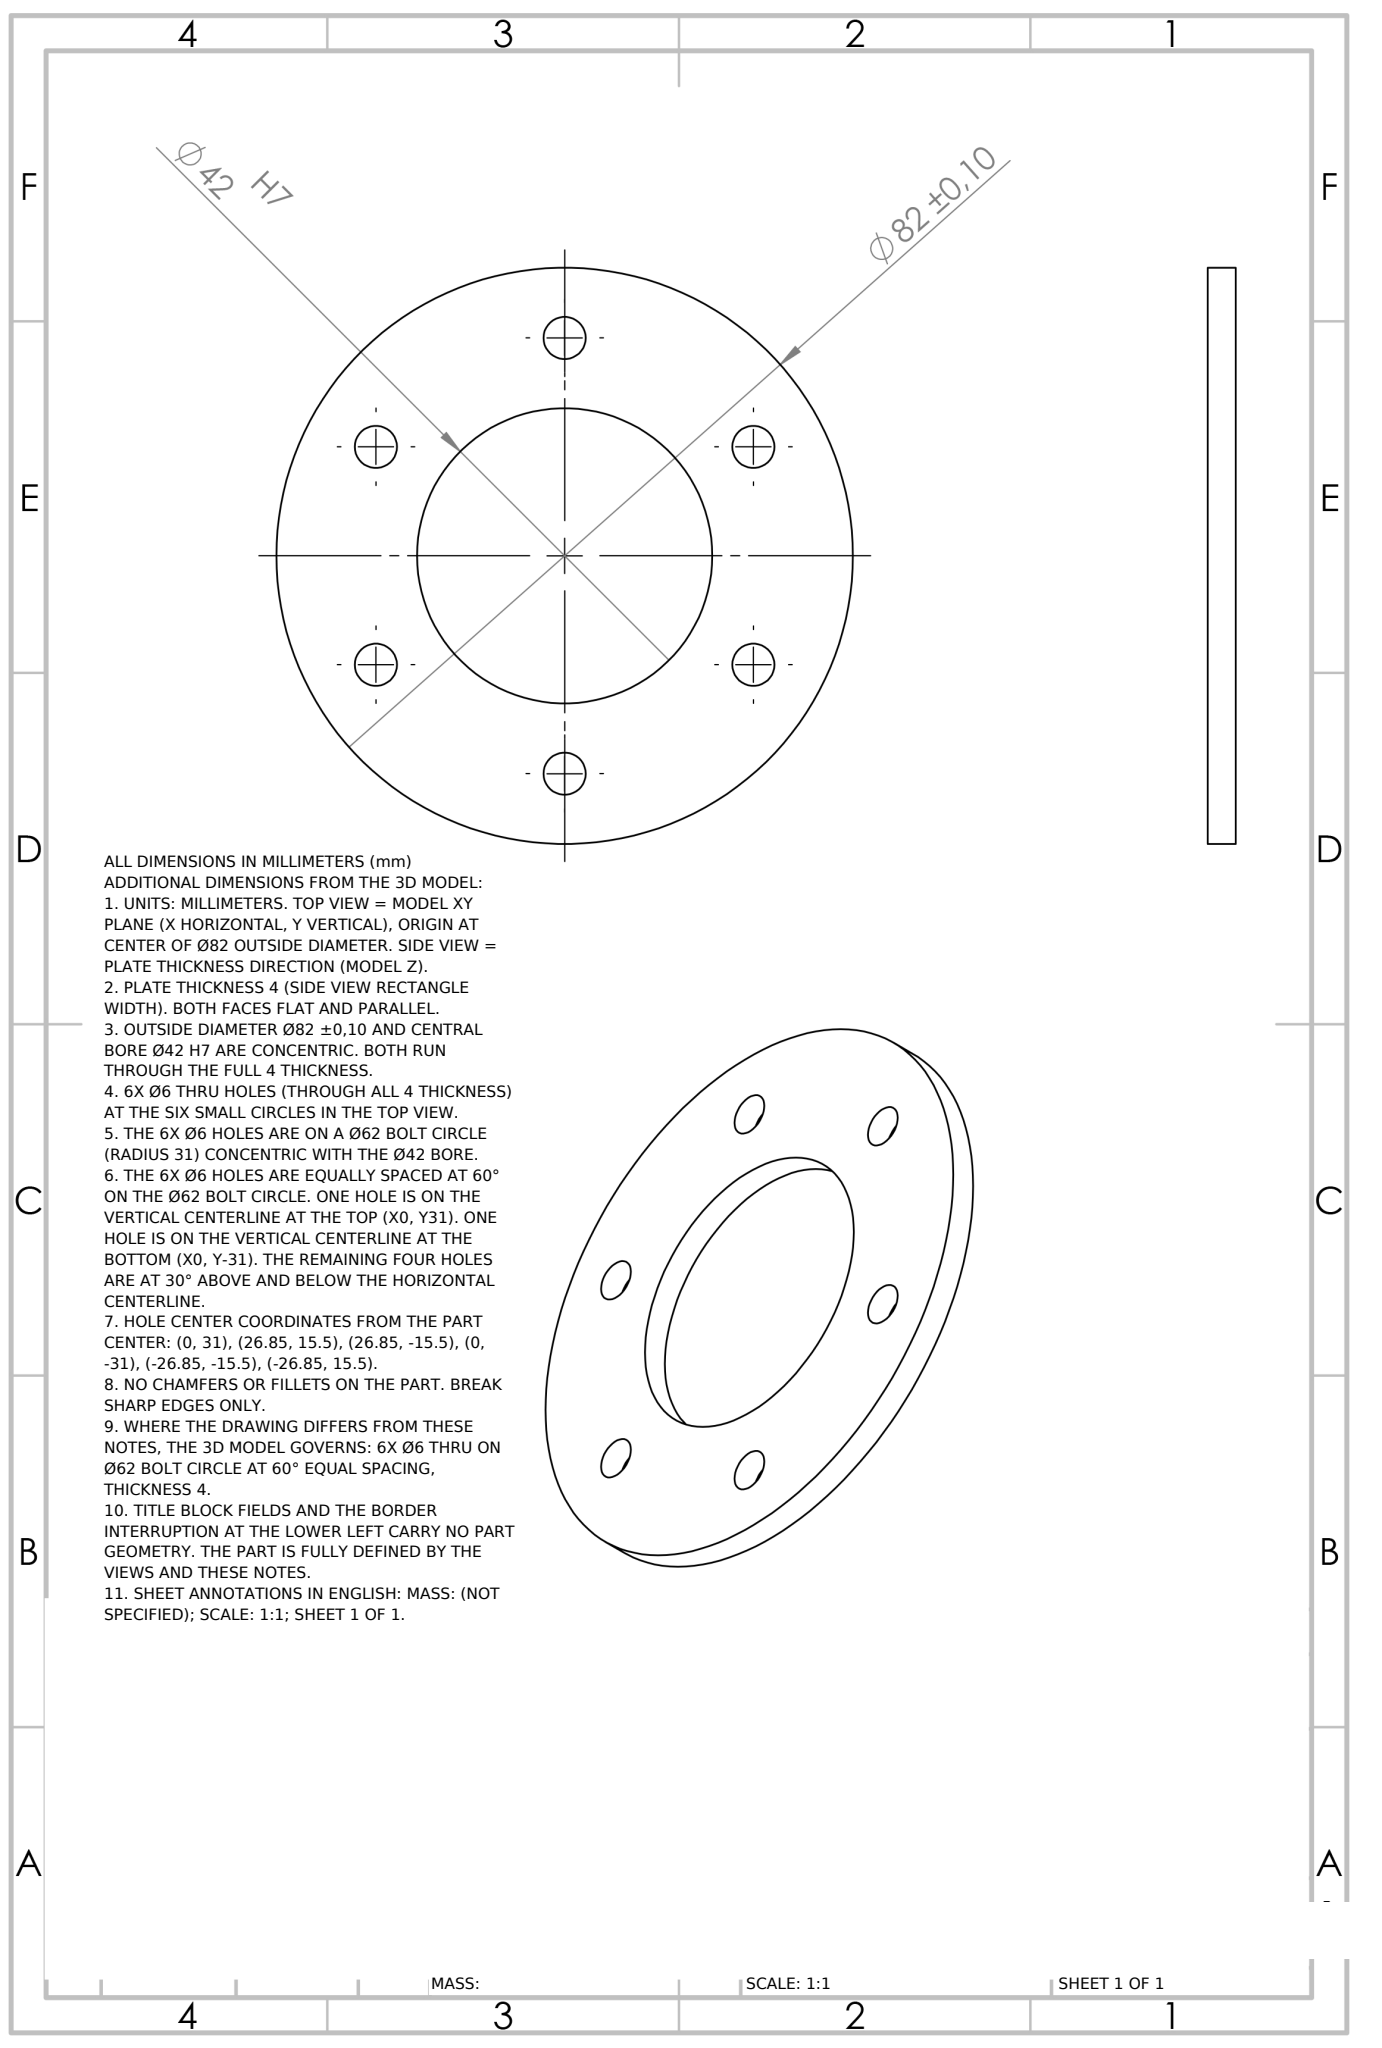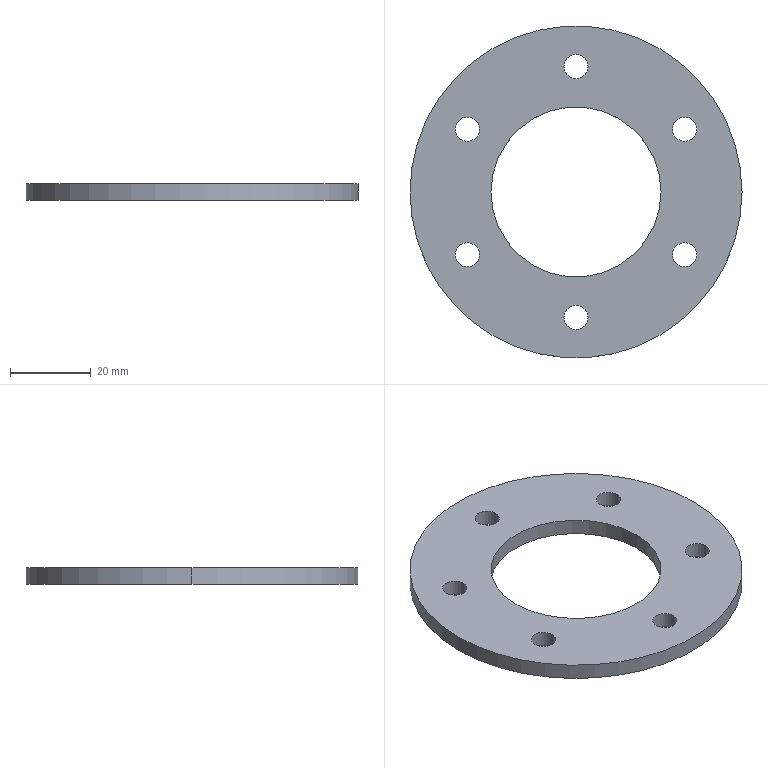Part | NX | mm | 1 solid | 18 faces | box 82 x 82 x 4 mm | volume 14904 mm3 | cylinder 16 | plane 2 | commonest cylinder face diameters 6 x12 42 x2 82 x2
STEP:
#1=COLOUR_RGB('',0.7922,0.8196,0.9333);
#2=FILL_AREA_STYLE_COLOUR('',#1);
#3=FILL_AREA_STYLE('',(#2));
#4=SURFACE_STYLE_FILL_AREA(#3);
#5=SURFACE_SIDE_STYLE('',(#4));
#6=SURFACE_STYLE_USAGE(.BOTH.,#5);
#7=PRESENTATION_STYLE_ASSIGNMENT((#6));
#8=CARTESIAN_POINT('',(-29.847,15.5,4.));
#9=VERTEX_POINT('',#8);
#10=CARTESIAN_POINT('',(-23.847,15.5,4.));
#11=VERTEX_POINT('',#10);
#12=CARTESIAN_POINT('',(-26.847,15.5,4.));
#13=DIRECTION('',(0.,0.,1.));
#14=DIRECTION('',(1.,0.,0.));
#15=AXIS2_PLACEMENT_3D('',#12,#13,#14);
#16=CIRCLE('',#15,3.);
#17=EDGE_CURVE('',#9,#11,#16,.T.);
#18=ORIENTED_EDGE('',*,*,#17,.T.);
#19=CARTESIAN_POINT('',(-23.847,15.5,0.));
#20=VERTEX_POINT('',#19);
#21=CARTESIAN_POINT('',(-23.847,15.5,4.));
#22=DIRECTION('',(0.,0.,-1.));
#23=VECTOR('',#22,1000.);
#24=LINE('',#21,#23);
#25=EDGE_CURVE('',#11,#20,#24,.T.);
#26=ORIENTED_EDGE('',*,*,#25,.T.);
#27=CARTESIAN_POINT('',(-29.847,15.5,0.));
#28=VERTEX_POINT('',#27);
#29=CARTESIAN_POINT('',(-26.847,15.5,0.));
#30=DIRECTION('',(0.,0.,1.));
#31=DIRECTION('',(1.,0.,0.));
#32=AXIS2_PLACEMENT_3D('',#29,#30,#31);
#33=CIRCLE('',#32,3.);
#34=EDGE_CURVE('',#28,#20,#33,.T.);
#35=ORIENTED_EDGE('',*,*,#34,.F.);
#36=CARTESIAN_POINT('',(-29.847,15.5,4.));
#37=DIRECTION('',(0.,0.,-1.));
#38=VECTOR('',#37,1000.);
#39=LINE('',#36,#38);
#40=EDGE_CURVE('',#9,#28,#39,.T.);
#41=ORIENTED_EDGE('',*,*,#40,.F.);
#42=EDGE_LOOP('',(#18,#26,#35,#41));
#43=FACE_OUTER_BOUND('',#42,.T.);
#44=CARTESIAN_POINT('',(-26.847,15.5,4.));
#45=DIRECTION('',(0.,0.,-1.));
#46=DIRECTION('',(-1.,0.,0.));
#47=AXIS2_PLACEMENT_3D('',#44,#45,#46);
#48=CYLINDRICAL_SURFACE('',#47,3.);
#49=ADVANCED_FACE('',(#43),#48,.F.);
#50=CARTESIAN_POINT('',(-29.847,-15.5,4.));
#51=VERTEX_POINT('',#50);
#52=CARTESIAN_POINT('',(-23.847,-15.5,4.));
#53=VERTEX_POINT('',#52);
#54=CARTESIAN_POINT('',(-26.847,-15.5,4.));
#55=DIRECTION('',(0.,0.,1.));
#56=DIRECTION('',(1.,0.,0.));
#57=AXIS2_PLACEMENT_3D('',#54,#55,#56);
#58=CIRCLE('',#57,3.);
#59=EDGE_CURVE('',#51,#53,#58,.T.);
#60=ORIENTED_EDGE('',*,*,#59,.T.);
#61=CARTESIAN_POINT('',(-23.847,-15.5,0.));
#62=VERTEX_POINT('',#61);
#63=CARTESIAN_POINT('',(-23.847,-15.5,4.));
#64=DIRECTION('',(0.,0.,-1.));
#65=VECTOR('',#64,1000.);
#66=LINE('',#63,#65);
#67=EDGE_CURVE('',#53,#62,#66,.T.);
#68=ORIENTED_EDGE('',*,*,#67,.T.);
#69=CARTESIAN_POINT('',(-29.847,-15.5,0.));
#70=VERTEX_POINT('',#69);
#71=CARTESIAN_POINT('',(-26.847,-15.5,0.));
#72=DIRECTION('',(0.,0.,1.));
#73=DIRECTION('',(1.,0.,0.));
#74=AXIS2_PLACEMENT_3D('',#71,#72,#73);
#75=CIRCLE('',#74,3.);
#76=EDGE_CURVE('',#70,#62,#75,.T.);
#77=ORIENTED_EDGE('',*,*,#76,.F.);
#78=CARTESIAN_POINT('',(-29.847,-15.5,4.));
#79=DIRECTION('',(0.,0.,-1.));
#80=VECTOR('',#79,1000.);
#81=LINE('',#78,#80);
#82=EDGE_CURVE('',#51,#70,#81,.T.);
#83=ORIENTED_EDGE('',*,*,#82,.F.);
#84=EDGE_LOOP('',(#60,#68,#77,#83));
#85=FACE_OUTER_BOUND('',#84,.T.);
#86=CARTESIAN_POINT('',(-26.847,-15.5,4.));
#87=DIRECTION('',(0.,0.,-1.));
#88=DIRECTION('',(-1.,0.,0.));
#89=AXIS2_PLACEMENT_3D('',#86,#87,#88);
#90=CYLINDRICAL_SURFACE('',#89,3.);
#91=ADVANCED_FACE('',(#85),#90,.F.);
#92=CARTESIAN_POINT('',(-3.,-31.,4.));
#93=VERTEX_POINT('',#92);
#94=CARTESIAN_POINT('',(3.,-31.,4.));
#95=VERTEX_POINT('',#94);
#96=CARTESIAN_POINT('',(0.,-31.,4.));
#97=DIRECTION('',(0.,0.,1.));
#98=DIRECTION('',(1.,0.,0.));
#99=AXIS2_PLACEMENT_3D('',#96,#97,#98);
#100=CIRCLE('',#99,3.);
#101=EDGE_CURVE('',#93,#95,#100,.T.);
#102=ORIENTED_EDGE('',*,*,#101,.T.);
#103=CARTESIAN_POINT('',(3.,-31.,0.));
#104=VERTEX_POINT('',#103);
#105=CARTESIAN_POINT('',(3.,-31.,4.));
#106=DIRECTION('',(0.,0.,-1.));
#107=VECTOR('',#106,1000.);
#108=LINE('',#105,#107);
#109=EDGE_CURVE('',#95,#104,#108,.T.);
#110=ORIENTED_EDGE('',*,*,#109,.T.);
#111=CARTESIAN_POINT('',(-3.,-31.,0.));
#112=VERTEX_POINT('',#111);
#113=CARTESIAN_POINT('',(0.,-31.,0.));
#114=DIRECTION('',(0.,0.,1.));
#115=DIRECTION('',(1.,0.,0.));
#116=AXIS2_PLACEMENT_3D('',#113,#114,#115);
#117=CIRCLE('',#116,3.);
#118=EDGE_CURVE('',#112,#104,#117,.T.);
#119=ORIENTED_EDGE('',*,*,#118,.F.);
#120=CARTESIAN_POINT('',(-3.,-31.,4.));
#121=DIRECTION('',(0.,0.,-1.));
#122=VECTOR('',#121,1000.);
#123=LINE('',#120,#122);
#124=EDGE_CURVE('',#93,#112,#123,.T.);
#125=ORIENTED_EDGE('',*,*,#124,.F.);
#126=EDGE_LOOP('',(#102,#110,#119,#125));
#127=FACE_OUTER_BOUND('',#126,.T.);
#128=CARTESIAN_POINT('',(0.,-31.,4.));
#129=DIRECTION('',(0.,0.,-1.));
#130=DIRECTION('',(-1.,0.,0.));
#131=AXIS2_PLACEMENT_3D('',#128,#129,#130);
#132=CYLINDRICAL_SURFACE('',#131,3.);
#133=ADVANCED_FACE('',(#127),#132,.F.);
#134=CARTESIAN_POINT('',(23.847,-15.5,4.));
#135=VERTEX_POINT('',#134);
#136=CARTESIAN_POINT('',(29.847,-15.5,4.));
#137=VERTEX_POINT('',#136);
#138=CARTESIAN_POINT('',(26.847,-15.5,4.));
#139=DIRECTION('',(0.,0.,1.));
#140=DIRECTION('',(1.,0.,0.));
#141=AXIS2_PLACEMENT_3D('',#138,#139,#140);
#142=CIRCLE('',#141,3.);
#143=EDGE_CURVE('',#135,#137,#142,.T.);
#144=ORIENTED_EDGE('',*,*,#143,.T.);
#145=CARTESIAN_POINT('',(29.847,-15.5,0.));
#146=VERTEX_POINT('',#145);
#147=CARTESIAN_POINT('',(29.847,-15.5,4.));
#148=DIRECTION('',(0.,0.,-1.));
#149=VECTOR('',#148,1000.);
#150=LINE('',#147,#149);
#151=EDGE_CURVE('',#137,#146,#150,.T.);
#152=ORIENTED_EDGE('',*,*,#151,.T.);
#153=CARTESIAN_POINT('',(23.847,-15.5,0.));
#154=VERTEX_POINT('',#153);
#155=CARTESIAN_POINT('',(26.847,-15.5,0.));
#156=DIRECTION('',(0.,0.,1.));
#157=DIRECTION('',(1.,0.,0.));
#158=AXIS2_PLACEMENT_3D('',#155,#156,#157);
#159=CIRCLE('',#158,3.);
#160=EDGE_CURVE('',#154,#146,#159,.T.);
#161=ORIENTED_EDGE('',*,*,#160,.F.);
#162=CARTESIAN_POINT('',(23.847,-15.5,4.));
#163=DIRECTION('',(0.,0.,-1.));
#164=VECTOR('',#163,1000.);
#165=LINE('',#162,#164);
#166=EDGE_CURVE('',#135,#154,#165,.T.);
#167=ORIENTED_EDGE('',*,*,#166,.F.);
#168=EDGE_LOOP('',(#144,#152,#161,#167));
#169=FACE_OUTER_BOUND('',#168,.T.);
#170=CARTESIAN_POINT('',(26.847,-15.5,4.));
#171=DIRECTION('',(0.,0.,-1.));
#172=DIRECTION('',(-1.,0.,0.));
#173=AXIS2_PLACEMENT_3D('',#170,#171,#172);
#174=CYLINDRICAL_SURFACE('',#173,3.);
#175=ADVANCED_FACE('',(#169),#174,.F.);
#176=CARTESIAN_POINT('',(23.847,15.5,4.));
#177=VERTEX_POINT('',#176);
#178=CARTESIAN_POINT('',(29.847,15.5,4.));
#179=VERTEX_POINT('',#178);
#180=CARTESIAN_POINT('',(26.847,15.5,4.));
#181=DIRECTION('',(0.,0.,1.));
#182=DIRECTION('',(1.,0.,0.));
#183=AXIS2_PLACEMENT_3D('',#180,#181,#182);
#184=CIRCLE('',#183,3.);
#185=EDGE_CURVE('',#177,#179,#184,.T.);
#186=ORIENTED_EDGE('',*,*,#185,.T.);
#187=CARTESIAN_POINT('',(29.847,15.5,0.));
#188=VERTEX_POINT('',#187);
#189=CARTESIAN_POINT('',(29.847,15.5,4.));
#190=DIRECTION('',(0.,0.,-1.));
#191=VECTOR('',#190,1000.);
#192=LINE('',#189,#191);
#193=EDGE_CURVE('',#179,#188,#192,.T.);
#194=ORIENTED_EDGE('',*,*,#193,.T.);
#195=CARTESIAN_POINT('',(23.847,15.5,0.));
#196=VERTEX_POINT('',#195);
#197=CARTESIAN_POINT('',(26.847,15.5,0.));
#198=DIRECTION('',(0.,0.,1.));
#199=DIRECTION('',(1.,0.,0.));
#200=AXIS2_PLACEMENT_3D('',#197,#198,#199);
#201=CIRCLE('',#200,3.);
#202=EDGE_CURVE('',#196,#188,#201,.T.);
#203=ORIENTED_EDGE('',*,*,#202,.F.);
#204=CARTESIAN_POINT('',(23.847,15.5,4.));
#205=DIRECTION('',(0.,0.,-1.));
#206=VECTOR('',#205,1000.);
#207=LINE('',#204,#206);
#208=EDGE_CURVE('',#177,#196,#207,.T.);
#209=ORIENTED_EDGE('',*,*,#208,.F.);
#210=EDGE_LOOP('',(#186,#194,#203,#209));
#211=FACE_OUTER_BOUND('',#210,.T.);
#212=CARTESIAN_POINT('',(26.847,15.5,4.));
#213=DIRECTION('',(0.,0.,-1.));
#214=DIRECTION('',(-1.,0.,0.));
#215=AXIS2_PLACEMENT_3D('',#212,#213,#214);
#216=CYLINDRICAL_SURFACE('',#215,3.);
#217=ADVANCED_FACE('',(#211),#216,.F.);
#218=CARTESIAN_POINT('',(-3.,31.,4.));
#219=VERTEX_POINT('',#218);
#220=CARTESIAN_POINT('',(3.,31.,4.));
#221=VERTEX_POINT('',#220);
#222=CARTESIAN_POINT('',(0.,31.,4.));
#223=DIRECTION('',(0.,0.,1.));
#224=DIRECTION('',(1.,0.,0.));
#225=AXIS2_PLACEMENT_3D('',#222,#223,#224);
#226=CIRCLE('',#225,3.);
#227=EDGE_CURVE('',#219,#221,#226,.T.);
#228=ORIENTED_EDGE('',*,*,#227,.T.);
#229=CARTESIAN_POINT('',(3.,31.,0.));
#230=VERTEX_POINT('',#229);
#231=CARTESIAN_POINT('',(3.,31.,4.));
#232=DIRECTION('',(0.,0.,-1.));
#233=VECTOR('',#232,1000.);
#234=LINE('',#231,#233);
#235=EDGE_CURVE('',#221,#230,#234,.T.);
#236=ORIENTED_EDGE('',*,*,#235,.T.);
#237=CARTESIAN_POINT('',(-3.,31.,0.));
#238=VERTEX_POINT('',#237);
#239=CARTESIAN_POINT('',(0.,31.,0.));
#240=DIRECTION('',(0.,0.,1.));
#241=DIRECTION('',(1.,0.,0.));
#242=AXIS2_PLACEMENT_3D('',#239,#240,#241);
#243=CIRCLE('',#242,3.);
#244=EDGE_CURVE('',#238,#230,#243,.T.);
#245=ORIENTED_EDGE('',*,*,#244,.F.);
#246=CARTESIAN_POINT('',(-3.,31.,4.));
#247=DIRECTION('',(0.,0.,-1.));
#248=VECTOR('',#247,1000.);
#249=LINE('',#246,#248);
#250=EDGE_CURVE('',#219,#238,#249,.T.);
#251=ORIENTED_EDGE('',*,*,#250,.F.);
#252=EDGE_LOOP('',(#228,#236,#245,#251));
#253=FACE_OUTER_BOUND('',#252,.T.);
#254=CARTESIAN_POINT('',(0.,31.,4.));
#255=DIRECTION('',(0.,0.,-1.));
#256=DIRECTION('',(-1.,0.,0.));
#257=AXIS2_PLACEMENT_3D('',#254,#255,#256);
#258=CYLINDRICAL_SURFACE('',#257,3.);
#259=ADVANCED_FACE('',(#253),#258,.F.);
#260=CARTESIAN_POINT('',(-21.,0.,4.));
#261=VERTEX_POINT('',#260);
#262=CARTESIAN_POINT('',(21.,0.,4.));
#263=VERTEX_POINT('',#262);
#264=CARTESIAN_POINT('',(0.,0.,4.));
#265=DIRECTION('',(0.,0.,1.));
#266=DIRECTION('',(1.,0.,0.));
#267=AXIS2_PLACEMENT_3D('',#264,#265,#266);
#268=CIRCLE('',#267,21.);
#269=EDGE_CURVE('',#261,#263,#268,.T.);
#270=ORIENTED_EDGE('',*,*,#269,.T.);
#271=CARTESIAN_POINT('',(21.,0.,0.));
#272=VERTEX_POINT('',#271);
#273=CARTESIAN_POINT('',(21.,0.,4.));
#274=DIRECTION('',(0.,0.,-1.));
#275=VECTOR('',#274,1000.);
#276=LINE('',#273,#275);
#277=EDGE_CURVE('',#263,#272,#276,.T.);
#278=ORIENTED_EDGE('',*,*,#277,.T.);
#279=CARTESIAN_POINT('',(-21.,0.,0.));
#280=VERTEX_POINT('',#279);
#281=CARTESIAN_POINT('',(0.,0.,0.));
#282=DIRECTION('',(0.,0.,1.));
#283=DIRECTION('',(1.,0.,0.));
#284=AXIS2_PLACEMENT_3D('',#281,#282,#283);
#285=CIRCLE('',#284,21.);
#286=EDGE_CURVE('',#280,#272,#285,.T.);
#287=ORIENTED_EDGE('',*,*,#286,.F.);
#288=CARTESIAN_POINT('',(-21.,0.,4.));
#289=DIRECTION('',(0.,0.,-1.));
#290=VECTOR('',#289,1000.);
#291=LINE('',#288,#290);
#292=EDGE_CURVE('',#261,#280,#291,.T.);
#293=ORIENTED_EDGE('',*,*,#292,.F.);
#294=EDGE_LOOP('',(#270,#278,#287,#293));
#295=FACE_OUTER_BOUND('',#294,.T.);
#296=CARTESIAN_POINT('',(0.,0.,4.));
#297=DIRECTION('',(0.,0.,-1.));
#298=DIRECTION('',(-1.,0.,0.));
#299=AXIS2_PLACEMENT_3D('',#296,#297,#298);
#300=CYLINDRICAL_SURFACE('',#299,21.);
#301=ADVANCED_FACE('',(#295),#300,.F.);
#302=CARTESIAN_POINT('',(41.,0.,4.));
#303=VERTEX_POINT('',#302);
#304=CARTESIAN_POINT('',(-41.,0.,4.));
#305=VERTEX_POINT('',#304);
#306=CARTESIAN_POINT('',(0.,0.,4.));
#307=DIRECTION('',(0.,0.,1.));
#308=DIRECTION('',(1.,0.,0.));
#309=AXIS2_PLACEMENT_3D('',#306,#307,#308);
#310=CIRCLE('',#309,41.);
#311=EDGE_CURVE('',#303,#305,#310,.T.);
#312=ORIENTED_EDGE('',*,*,#311,.F.);
#313=CARTESIAN_POINT('',(41.,0.,0.));
#314=VERTEX_POINT('',#313);
#315=CARTESIAN_POINT('',(41.,0.,4.));
#316=DIRECTION('',(0.,0.,-1.));
#317=VECTOR('',#316,1000.);
#318=LINE('',#315,#317);
#319=EDGE_CURVE('',#303,#314,#318,.T.);
#320=ORIENTED_EDGE('',*,*,#319,.T.);
#321=CARTESIAN_POINT('',(-41.,0.,0.));
#322=VERTEX_POINT('',#321);
#323=CARTESIAN_POINT('',(0.,0.,0.));
#324=DIRECTION('',(0.,0.,1.));
#325=DIRECTION('',(1.,0.,0.));
#326=AXIS2_PLACEMENT_3D('',#323,#324,#325);
#327=CIRCLE('',#326,41.);
#328=EDGE_CURVE('',#314,#322,#327,.T.);
#329=ORIENTED_EDGE('',*,*,#328,.T.);
#330=CARTESIAN_POINT('',(-41.,0.,4.));
#331=DIRECTION('',(0.,0.,-1.));
#332=VECTOR('',#331,1000.);
#333=LINE('',#330,#332);
#334=EDGE_CURVE('',#305,#322,#333,.T.);
#335=ORIENTED_EDGE('',*,*,#334,.F.);
#336=EDGE_LOOP('',(#312,#320,#329,#335));
#337=FACE_OUTER_BOUND('',#336,.T.);
#338=CARTESIAN_POINT('',(0.,0.,4.));
#339=DIRECTION('',(0.,0.,-1.));
#340=DIRECTION('',(-1.,0.,0.));
#341=AXIS2_PLACEMENT_3D('',#338,#339,#340);
#342=CYLINDRICAL_SURFACE('',#341,41.);
#343=ADVANCED_FACE('',(#337),#342,.T.);
#344=ORIENTED_EDGE('',*,*,#59,.F.);
#345=CARTESIAN_POINT('',(-26.847,-15.5,4.));
#346=DIRECTION('',(0.,0.,1.));
#347=DIRECTION('',(1.,0.,0.));
#348=AXIS2_PLACEMENT_3D('',#345,#346,#347);
#349=CIRCLE('',#348,3.);
#350=EDGE_CURVE('',#53,#51,#349,.T.);
#351=ORIENTED_EDGE('',*,*,#350,.F.);
#352=EDGE_LOOP('',(#344,#351));
#353=FACE_BOUND('',#352,.T.);
#354=ORIENTED_EDGE('',*,*,#143,.F.);
#355=CARTESIAN_POINT('',(26.847,-15.5,4.));
#356=DIRECTION('',(0.,0.,1.));
#357=DIRECTION('',(1.,0.,0.));
#358=AXIS2_PLACEMENT_3D('',#355,#356,#357);
#359=CIRCLE('',#358,3.);
#360=EDGE_CURVE('',#137,#135,#359,.T.);
#361=ORIENTED_EDGE('',*,*,#360,.F.);
#362=EDGE_LOOP('',(#354,#361));
#363=FACE_BOUND('',#362,.T.);
#364=ORIENTED_EDGE('',*,*,#227,.F.);
#365=CARTESIAN_POINT('',(0.,31.,4.));
#366=DIRECTION('',(0.,0.,1.));
#367=DIRECTION('',(1.,0.,0.));
#368=AXIS2_PLACEMENT_3D('',#365,#366,#367);
#369=CIRCLE('',#368,3.);
#370=EDGE_CURVE('',#221,#219,#369,.T.);
#371=ORIENTED_EDGE('',*,*,#370,.F.);
#372=EDGE_LOOP('',(#364,#371));
#373=FACE_BOUND('',#372,.T.);
#374=CARTESIAN_POINT('',(0.,0.,4.));
#375=DIRECTION('',(0.,0.,1.));
#376=DIRECTION('',(1.,0.,0.));
#377=AXIS2_PLACEMENT_3D('',#374,#375,#376);
#378=CIRCLE('',#377,41.);
#379=EDGE_CURVE('',#305,#303,#378,.T.);
#380=ORIENTED_EDGE('',*,*,#379,.T.);
#381=ORIENTED_EDGE('',*,*,#311,.T.);
#382=EDGE_LOOP('',(#380,#381));
#383=FACE_OUTER_BOUND('',#382,.T.);
#384=ORIENTED_EDGE('',*,*,#269,.F.);
#385=CARTESIAN_POINT('',(0.,0.,4.));
#386=DIRECTION('',(0.,0.,1.));
#387=DIRECTION('',(1.,0.,0.));
#388=AXIS2_PLACEMENT_3D('',#385,#386,#387);
#389=CIRCLE('',#388,21.);
#390=EDGE_CURVE('',#263,#261,#389,.T.);
#391=ORIENTED_EDGE('',*,*,#390,.F.);
#392=EDGE_LOOP('',(#384,#391));
#393=FACE_BOUND('',#392,.T.);
#394=ORIENTED_EDGE('',*,*,#185,.F.);
#395=CARTESIAN_POINT('',(26.847,15.5,4.));
#396=DIRECTION('',(0.,0.,1.));
#397=DIRECTION('',(1.,0.,0.));
#398=AXIS2_PLACEMENT_3D('',#395,#396,#397);
#399=CIRCLE('',#398,3.);
#400=EDGE_CURVE('',#179,#177,#399,.T.);
#401=ORIENTED_EDGE('',*,*,#400,.F.);
#402=EDGE_LOOP('',(#394,#401));
#403=FACE_BOUND('',#402,.T.);
#404=ORIENTED_EDGE('',*,*,#101,.F.);
#405=CARTESIAN_POINT('',(0.,-31.,4.));
#406=DIRECTION('',(0.,0.,1.));
#407=DIRECTION('',(1.,0.,0.));
#408=AXIS2_PLACEMENT_3D('',#405,#406,#407);
#409=CIRCLE('',#408,3.);
#410=EDGE_CURVE('',#95,#93,#409,.T.);
#411=ORIENTED_EDGE('',*,*,#410,.F.);
#412=EDGE_LOOP('',(#404,#411));
#413=FACE_BOUND('',#412,.T.);
#414=ORIENTED_EDGE('',*,*,#17,.F.);
#415=CARTESIAN_POINT('',(-26.847,15.5,4.));
#416=DIRECTION('',(0.,0.,1.));
#417=DIRECTION('',(1.,0.,0.));
#418=AXIS2_PLACEMENT_3D('',#415,#416,#417);
#419=CIRCLE('',#418,3.);
#420=EDGE_CURVE('',#11,#9,#419,.T.);
#421=ORIENTED_EDGE('',*,*,#420,.F.);
#422=EDGE_LOOP('',(#414,#421));
#423=FACE_BOUND('',#422,.T.);
#424=CARTESIAN_POINT('',(0.,0.,4.));
#425=DIRECTION('',(0.,0.,1.));
#426=DIRECTION('',(1.,0.,0.));
#427=AXIS2_PLACEMENT_3D('',#424,#425,#426);
#428=PLANE('',#427);
#429=ADVANCED_FACE('',(#353,#363,#373,#383,#393,#403,#413,#423),#428,.T.);
#430=CARTESIAN_POINT('',(0.,0.,0.));
#431=DIRECTION('',(0.,0.,1.));
#432=DIRECTION('',(1.,0.,0.));
#433=AXIS2_PLACEMENT_3D('',#430,#431,#432);
#434=CIRCLE('',#433,41.);
#435=EDGE_CURVE('',#322,#314,#434,.T.);
#436=ORIENTED_EDGE('',*,*,#435,.F.);
#437=ORIENTED_EDGE('',*,*,#328,.F.);
#438=EDGE_LOOP('',(#436,#437));
#439=FACE_OUTER_BOUND('',#438,.T.);
#440=ORIENTED_EDGE('',*,*,#286,.T.);
#441=CARTESIAN_POINT('',(0.,0.,0.));
#442=DIRECTION('',(0.,0.,1.));
#443=DIRECTION('',(1.,0.,0.));
#444=AXIS2_PLACEMENT_3D('',#441,#442,#443);
#445=CIRCLE('',#444,21.);
#446=EDGE_CURVE('',#272,#280,#445,.T.);
#447=ORIENTED_EDGE('',*,*,#446,.T.);
#448=EDGE_LOOP('',(#440,#447));
#449=FACE_BOUND('',#448,.T.);
#450=ORIENTED_EDGE('',*,*,#244,.T.);
#451=CARTESIAN_POINT('',(0.,31.,0.));
#452=DIRECTION('',(0.,0.,1.));
#453=DIRECTION('',(1.,0.,0.));
#454=AXIS2_PLACEMENT_3D('',#451,#452,#453);
#455=CIRCLE('',#454,3.);
#456=EDGE_CURVE('',#230,#238,#455,.T.);
#457=ORIENTED_EDGE('',*,*,#456,.T.);
#458=EDGE_LOOP('',(#450,#457));
#459=FACE_BOUND('',#458,.T.);
#460=ORIENTED_EDGE('',*,*,#202,.T.);
#461=CARTESIAN_POINT('',(26.847,15.5,0.));
#462=DIRECTION('',(0.,0.,1.));
#463=DIRECTION('',(1.,0.,0.));
#464=AXIS2_PLACEMENT_3D('',#461,#462,#463);
#465=CIRCLE('',#464,3.);
#466=EDGE_CURVE('',#188,#196,#465,.T.);
#467=ORIENTED_EDGE('',*,*,#466,.T.);
#468=EDGE_LOOP('',(#460,#467));
#469=FACE_BOUND('',#468,.T.);
#470=ORIENTED_EDGE('',*,*,#160,.T.);
#471=CARTESIAN_POINT('',(26.847,-15.5,0.));
#472=DIRECTION('',(0.,0.,1.));
#473=DIRECTION('',(1.,0.,0.));
#474=AXIS2_PLACEMENT_3D('',#471,#472,#473);
#475=CIRCLE('',#474,3.);
#476=EDGE_CURVE('',#146,#154,#475,.T.);
#477=ORIENTED_EDGE('',*,*,#476,.T.);
#478=EDGE_LOOP('',(#470,#477));
#479=FACE_BOUND('',#478,.T.);
#480=ORIENTED_EDGE('',*,*,#118,.T.);
#481=CARTESIAN_POINT('',(0.,-31.,0.));
#482=DIRECTION('',(0.,0.,1.));
#483=DIRECTION('',(1.,0.,0.));
#484=AXIS2_PLACEMENT_3D('',#481,#482,#483);
#485=CIRCLE('',#484,3.);
#486=EDGE_CURVE('',#104,#112,#485,.T.);
#487=ORIENTED_EDGE('',*,*,#486,.T.);
#488=EDGE_LOOP('',(#480,#487));
#489=FACE_BOUND('',#488,.T.);
#490=ORIENTED_EDGE('',*,*,#76,.T.);
#491=CARTESIAN_POINT('',(-26.847,-15.5,0.));
#492=DIRECTION('',(0.,0.,1.));
#493=DIRECTION('',(1.,0.,0.));
#494=AXIS2_PLACEMENT_3D('',#491,#492,#493);
#495=CIRCLE('',#494,3.);
#496=EDGE_CURVE('',#62,#70,#495,.T.);
#497=ORIENTED_EDGE('',*,*,#496,.T.);
#498=EDGE_LOOP('',(#490,#497));
#499=FACE_BOUND('',#498,.T.);
#500=ORIENTED_EDGE('',*,*,#34,.T.);
#501=CARTESIAN_POINT('',(-26.847,15.5,0.));
#502=DIRECTION('',(0.,0.,1.));
#503=DIRECTION('',(1.,0.,0.));
#504=AXIS2_PLACEMENT_3D('',#501,#502,#503);
#505=CIRCLE('',#504,3.);
#506=EDGE_CURVE('',#20,#28,#505,.T.);
#507=ORIENTED_EDGE('',*,*,#506,.T.);
#508=EDGE_LOOP('',(#500,#507));
#509=FACE_BOUND('',#508,.T.);
#510=CARTESIAN_POINT('',(0.,0.,0.));
#511=DIRECTION('',(0.,0.,1.));
#512=DIRECTION('',(1.,0.,0.));
#513=AXIS2_PLACEMENT_3D('',#510,#511,#512);
#514=PLANE('',#513);
#515=ADVANCED_FACE('',(#439,#449,#459,#469,#479,#489,#499,#509),#514,.F.);
#516=ORIENTED_EDGE('',*,*,#319,.F.);
#517=ORIENTED_EDGE('',*,*,#379,.F.);
#518=ORIENTED_EDGE('',*,*,#334,.T.);
#519=ORIENTED_EDGE('',*,*,#435,.T.);
#520=EDGE_LOOP('',(#516,#517,#518,#519));
#521=FACE_OUTER_BOUND('',#520,.T.);
#522=CARTESIAN_POINT('',(0.,0.,4.));
#523=DIRECTION('',(0.,0.,-1.));
#524=DIRECTION('',(-1.,0.,0.));
#525=AXIS2_PLACEMENT_3D('',#522,#523,#524);
#526=CYLINDRICAL_SURFACE('',#525,41.);
#527=ADVANCED_FACE('',(#521),#526,.T.);
#528=ORIENTED_EDGE('',*,*,#277,.F.);
#529=ORIENTED_EDGE('',*,*,#390,.T.);
#530=ORIENTED_EDGE('',*,*,#292,.T.);
#531=ORIENTED_EDGE('',*,*,#446,.F.);
#532=EDGE_LOOP('',(#528,#529,#530,#531));
#533=FACE_OUTER_BOUND('',#532,.T.);
#534=CARTESIAN_POINT('',(0.,0.,4.));
#535=DIRECTION('',(0.,0.,-1.));
#536=DIRECTION('',(-1.,0.,0.));
#537=AXIS2_PLACEMENT_3D('',#534,#535,#536);
#538=CYLINDRICAL_SURFACE('',#537,21.);
#539=ADVANCED_FACE('',(#533),#538,.F.);
#540=ORIENTED_EDGE('',*,*,#235,.F.);
#541=ORIENTED_EDGE('',*,*,#370,.T.);
#542=ORIENTED_EDGE('',*,*,#250,.T.);
#543=ORIENTED_EDGE('',*,*,#456,.F.);
#544=EDGE_LOOP('',(#540,#541,#542,#543));
#545=FACE_OUTER_BOUND('',#544,.T.);
#546=CARTESIAN_POINT('',(0.,31.,4.));
#547=DIRECTION('',(0.,0.,-1.));
#548=DIRECTION('',(-1.,0.,0.));
#549=AXIS2_PLACEMENT_3D('',#546,#547,#548);
#550=CYLINDRICAL_SURFACE('',#549,3.);
#551=ADVANCED_FACE('',(#545),#550,.F.);
#552=ORIENTED_EDGE('',*,*,#193,.F.);
#553=ORIENTED_EDGE('',*,*,#400,.T.);
#554=ORIENTED_EDGE('',*,*,#208,.T.);
#555=ORIENTED_EDGE('',*,*,#466,.F.);
#556=EDGE_LOOP('',(#552,#553,#554,#555));
#557=FACE_OUTER_BOUND('',#556,.T.);
#558=CARTESIAN_POINT('',(26.847,15.5,4.));
#559=DIRECTION('',(0.,0.,-1.));
#560=DIRECTION('',(-1.,0.,0.));
#561=AXIS2_PLACEMENT_3D('',#558,#559,#560);
#562=CYLINDRICAL_SURFACE('',#561,3.);
#563=ADVANCED_FACE('',(#557),#562,.F.);
#564=ORIENTED_EDGE('',*,*,#151,.F.);
#565=ORIENTED_EDGE('',*,*,#360,.T.);
#566=ORIENTED_EDGE('',*,*,#166,.T.);
#567=ORIENTED_EDGE('',*,*,#476,.F.);
#568=EDGE_LOOP('',(#564,#565,#566,#567));
#569=FACE_OUTER_BOUND('',#568,.T.);
#570=CARTESIAN_POINT('',(26.847,-15.5,4.));
#571=DIRECTION('',(0.,0.,-1.));
#572=DIRECTION('',(-1.,0.,0.));
#573=AXIS2_PLACEMENT_3D('',#570,#571,#572);
#574=CYLINDRICAL_SURFACE('',#573,3.);
#575=ADVANCED_FACE('',(#569),#574,.F.);
#576=ORIENTED_EDGE('',*,*,#109,.F.);
#577=ORIENTED_EDGE('',*,*,#410,.T.);
#578=ORIENTED_EDGE('',*,*,#124,.T.);
#579=ORIENTED_EDGE('',*,*,#486,.F.);
#580=EDGE_LOOP('',(#576,#577,#578,#579));
#581=FACE_OUTER_BOUND('',#580,.T.);
#582=CARTESIAN_POINT('',(0.,-31.,4.));
#583=DIRECTION('',(0.,0.,-1.));
#584=DIRECTION('',(-1.,0.,0.));
#585=AXIS2_PLACEMENT_3D('',#582,#583,#584);
#586=CYLINDRICAL_SURFACE('',#585,3.);
#587=ADVANCED_FACE('',(#581),#586,.F.);
#588=ORIENTED_EDGE('',*,*,#67,.F.);
#589=ORIENTED_EDGE('',*,*,#350,.T.);
#590=ORIENTED_EDGE('',*,*,#82,.T.);
#591=ORIENTED_EDGE('',*,*,#496,.F.);
#592=EDGE_LOOP('',(#588,#589,#590,#591));
#593=FACE_OUTER_BOUND('',#592,.T.);
#594=CARTESIAN_POINT('',(-26.847,-15.5,4.));
#595=DIRECTION('',(0.,0.,-1.));
#596=DIRECTION('',(-1.,0.,0.));
#597=AXIS2_PLACEMENT_3D('',#594,#595,#596);
#598=CYLINDRICAL_SURFACE('',#597,3.);
#599=ADVANCED_FACE('',(#593),#598,.F.);
#600=ORIENTED_EDGE('',*,*,#25,.F.);
#601=ORIENTED_EDGE('',*,*,#420,.T.);
#602=ORIENTED_EDGE('',*,*,#40,.T.);
#603=ORIENTED_EDGE('',*,*,#506,.F.);
#604=EDGE_LOOP('',(#600,#601,#602,#603));
#605=FACE_OUTER_BOUND('',#604,.T.);
#606=CARTESIAN_POINT('',(-26.847,15.5,4.));
#607=DIRECTION('',(0.,0.,-1.));
#608=DIRECTION('',(-1.,0.,0.));
#609=AXIS2_PLACEMENT_3D('',#606,#607,#608);
#610=CYLINDRICAL_SURFACE('',#609,3.);
#611=ADVANCED_FACE('',(#605),#610,.F.);
#612=CLOSED_SHELL('',(#49,#91,#133,#175,#217,#259,#301,#343,#429,#515,#527,#539,#551,#563,#575,#587,#599,#611));
#613=MANIFOLD_SOLID_BREP('',#612);
#614=STYLED_ITEM('',(#7),#613);
#615=PRESENTATION_LAYER_ASSIGNMENT('','',(#614));
#616=COLOUR_RGB('',0.7922,0.8196,0.9333);
#617=FILL_AREA_STYLE_COLOUR('',#616);
#618=FILL_AREA_STYLE('',(#617));
#619=SURFACE_STYLE_FILL_AREA(#618);
#620=SURFACE_SIDE_STYLE('',(#619));
#621=SURFACE_STYLE_USAGE(.BOTH.,#620);
#622=PRESENTATION_STYLE_ASSIGNMENT((#621));
#623=CARTESIAN_POINT('',(0.,0.,0.));
#624=DIRECTION('',(0.,0.,1.));
#625=DIRECTION('',(1.,0.,0.));
#626=AXIS2_PLACEMENT_3D('',#623,#624,#625);
#627=(LENGTH_UNIT()NAMED_UNIT(*)SI_UNIT(.MILLI.,.METRE.));
#628=UNCERTAINTY_MEASURE_WITH_UNIT(LENGTH_MEASURE(0.00001),#627,'','');
#629=(NAMED_UNIT(*)PLANE_ANGLE_UNIT()SI_UNIT($,.RADIAN.));
#630=(NAMED_UNIT(*)SI_UNIT($,.STERADIAN.)SOLID_ANGLE_UNIT());
#631=(GEOMETRIC_REPRESENTATION_CONTEXT(3)GLOBAL_UNCERTAINTY_ASSIGNED_CONTEXT((#628))GLOBAL_UNIT_ASSIGNED_CONTEXT((#627,#629,#630))REPRESENTATION_CONTEXT('',''));
#632=ADVANCED_BREP_SHAPE_REPRESENTATION('',(#613,#626),#631);
#633=STYLED_ITEM('',(#622),#632);
#634=PRESENTATION_LAYER_ASSIGNMENT('','',(#633));
#635=(LENGTH_UNIT()NAMED_UNIT(*)SI_UNIT(.MILLI.,.METRE.));
#636=UNCERTAINTY_MEASURE_WITH_UNIT(LENGTH_MEASURE(0.00001),#635,'','');
#637=(NAMED_UNIT(*)PLANE_ANGLE_UNIT()SI_UNIT($,.RADIAN.));
#638=(NAMED_UNIT(*)SI_UNIT($,.STERADIAN.)SOLID_ANGLE_UNIT());
#639=(GEOMETRIC_REPRESENTATION_CONTEXT(3)GLOBAL_UNCERTAINTY_ASSIGNED_CONTEXT((#636))GLOBAL_UNIT_ASSIGNED_CONTEXT((#635,#637,#638))REPRESENTATION_CONTEXT('',''));
#640=MECHANICAL_DESIGN_GEOMETRIC_PRESENTATION_REPRESENTATION('',(#633),#639);
#641=(LENGTH_UNIT()NAMED_UNIT(*)SI_UNIT(.MILLI.,.METRE.));
#642=UNCERTAINTY_MEASURE_WITH_UNIT(LENGTH_MEASURE(0.00001),#641,'','');
#643=(NAMED_UNIT(*)PLANE_ANGLE_UNIT()SI_UNIT($,.RADIAN.));
#644=(NAMED_UNIT(*)SI_UNIT($,.STERADIAN.)SOLID_ANGLE_UNIT());
#645=(GEOMETRIC_REPRESENTATION_CONTEXT(3)GLOBAL_UNCERTAINTY_ASSIGNED_CONTEXT((#642))GLOBAL_UNIT_ASSIGNED_CONTEXT((#641,#643,#644))REPRESENTATION_CONTEXT('',''));
#646=MECHANICAL_DESIGN_GEOMETRIC_PRESENTATION_REPRESENTATION('',(#614),#645);